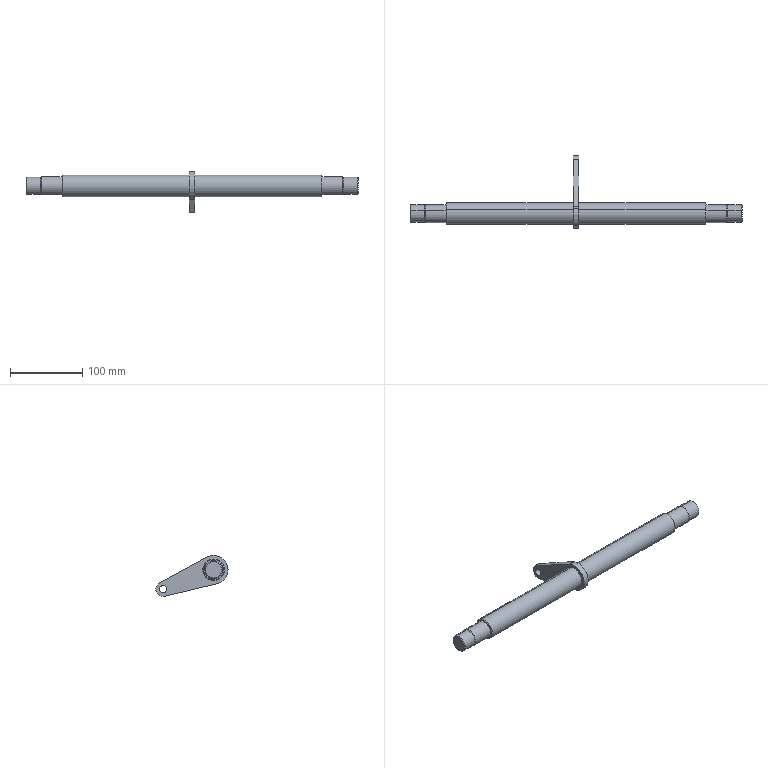Component | SolidWorks | OT-0100-005(RotatingShaft)-1 | 1 solid | 40 faces | box 460 x 99.97 x 57 mm | volume 319935 mm3 | cylinder 18 | cone 12 | plane 10 | commonest cylinder face diameters 30 x4 25 x4 24 x4 40 x3 10 x2 20 x1 | material Plain Carbon Steel
build123d program:
from build123d import *

# Parameters (mm, degrees)
SKETCH4_R           = 12
BOSS_EXTRUDE1_DEPTH = 20
BOSS_EXTRUDE2_START = 20
SKETCH5_R           = 12
BOSS_EXTRUDE2_DEPTH = 20
CHAMFER1_SIZE       = 1
SKETCH6_R           = 5
BOSS_EXTRUDE3_DEPTH = 4


with BuildPart() as part:
    # Sketch1 → Revolve1 (revolve)
    with BuildSketch(Plane(origin=(0, 0, 0), x_dir=(1, 0, 0), z_dir=(0, 1, 0))):
        Polygon((-210, 0), (-210, 11.5), (-209, 12.5), (-180, 12.5), (-180, 14), (-179, 15), (179, 15), (180, 14), (180, 12.5), (209, 12.5), (210, 11.5), (210, 0), align=None)
    revolve(axis=Axis((210, 0, 0), (-1, 0, 0)))

    # Sketch4 → Boss-Extrude1 (add)
    with BuildSketch(Plane(origin=(210, 0, 0), x_dir=(0, 0, -1), z_dir=(1, 0, 0))):
        Circle(SKETCH4_R)
    extrude(amount=BOSS_EXTRUDE1_DEPTH)

    # Sketch5 → Boss-Extrude2 (add)
    with BuildSketch(Plane.ZY.offset(210).offset(BOSS_EXTRUDE2_START)):
        with Locations(Location((0, 0, 0), (0, 0, 180))):
            Circle(SKETCH5_R)
    extrude(amount=-BOSS_EXTRUDE2_DEPTH)

    # Chamfer1
    chamfer1_edges = [part.edges().sort_by_distance(p)[0] for p in [
        (230, 0, 12),
        (-230, 0, 12),
    ]]
    chamfer(chamfer1_edges, length=CHAMFER1_SIZE)

    # Sketch6 → Boss-Extrude3 (add, symmetric)
    with BuildSketch(Plane(origin=(0, 0, 0), x_dir=(0, 0, -1), z_dir=(1, 0, 0))):
        with BuildLine():
            Line((-19.821, 2.667), (-9.911, 76.333))
            ThreePointArc((-9.911, 76.333), (0, 85), (9.911, 76.333))
            Line((9.911, 76.333), (19.821, 2.667))
            ThreePointArc((19.821, 2.667), (0, -20), (-19.821, 2.667))
        make_face()
        with Locations((0, 75)):
            Circle(SKETCH6_R, mode=Mode.SUBTRACT)
    extrude(amount=BOSS_EXTRUDE3_DEPTH, both=True)


solid = part.part

# Placed as in the assembly
solid = solid.moved(Location((200, 35, 0), (-21.097, 0, 0)))
STEP:
#1=COLOUR_RGB('',0.7922,0.8196,0.9333);
#2=FILL_AREA_STYLE_COLOUR('',#1);
#3=FILL_AREA_STYLE('',(#2));
#4=SURFACE_STYLE_FILL_AREA(#3);
#5=SURFACE_SIDE_STYLE('',(#4));
#6=SURFACE_STYLE_USAGE(.BOTH.,#5);
#7=PRESENTATION_STYLE_ASSIGNMENT((#6));
#8=CARTESIAN_POINT('',(8.031,1.591,0.551));
#9=VERTEX_POINT('',#8);
#10=CARTESIAN_POINT('',(8.031,1.165,-0.551));
#11=VERTEX_POINT('',#10);
#12=CARTESIAN_POINT('',(8.031,1.378,0.));
#13=DIRECTION('',(-1.,0.,0.));
#14=DIRECTION('',(0.,-0.3599,-0.933));
#15=AXIS2_PLACEMENT_3D('',#12,#13,#14);
#16=CIRCLE('',#15,0.5906);
#17=EDGE_CURVE('',#9,#11,#16,.T.);
#18=ORIENTED_EDGE('',*,*,#17,.F.);
#19=CARTESIAN_POINT('',(14.921,1.591,0.551));
#20=VERTEX_POINT('',#19);
#21=CARTESIAN_POINT('',(16.142,1.591,0.551));
#22=DIRECTION('',(1.,0.,0.));
#23=VECTOR('',#22,39.37);
#24=LINE('',#21,#23);
#25=EDGE_CURVE('',#9,#20,#24,.T.);
#26=ORIENTED_EDGE('',*,*,#25,.T.);
#27=CARTESIAN_POINT('',(14.921,1.165,-0.551));
#28=VERTEX_POINT('',#27);
#29=CARTESIAN_POINT('',(14.921,1.378,0.));
#30=DIRECTION('',(1.,0.,0.));
#31=DIRECTION('',(0.,-0.3599,-0.933));
#32=AXIS2_PLACEMENT_3D('',#29,#30,#31);
#33=CIRCLE('',#32,0.5906);
#34=EDGE_CURVE('',#28,#20,#33,.T.);
#35=ORIENTED_EDGE('',*,*,#34,.F.);
#36=CARTESIAN_POINT('',(16.142,1.165,-0.551));
#37=DIRECTION('',(1.,0.,0.));
#38=VECTOR('',#37,39.37);
#39=LINE('',#36,#38);
#40=EDGE_CURVE('',#11,#28,#39,.T.);
#41=ORIENTED_EDGE('',*,*,#40,.F.);
#42=EDGE_LOOP('',(#18,#26,#35,#41));
#43=FACE_OUTER_BOUND('',#42,.T.);
#44=CARTESIAN_POINT('',(16.142,1.378,0.));
#45=DIRECTION('',(1.,0.,0.));
#46=DIRECTION('',(0.,-0.3599,-0.933));
#47=AXIS2_PLACEMENT_3D('',#44,#45,#46);
#48=CYLINDRICAL_SURFACE('',#47,0.5906);
#49=ADVANCED_FACE('',(#43),#48,.T.);
#50=CARTESIAN_POINT('',(14.961,1.18,-0.5142));
#51=VERTEX_POINT('',#50);
#52=CARTESIAN_POINT('',(14.961,1.576,0.5142));
#53=VERTEX_POINT('',#52);
#54=CARTESIAN_POINT('',(14.961,1.378,0.));
#55=DIRECTION('',(1.,0.,0.));
#56=DIRECTION('',(0.,-0.3599,-0.933));
#57=AXIS2_PLACEMENT_3D('',#54,#55,#56);
#58=CIRCLE('',#57,0.5512);
#59=EDGE_CURVE('',#51,#53,#58,.T.);
#60=ORIENTED_EDGE('',*,*,#59,.F.);
#61=CARTESIAN_POINT('',(14.961,1.18,-0.5142));
#62=DIRECTION('',(-0.7071,-0.2545,-0.6597));
#63=VECTOR('',#62,39.37);
#64=LINE('',#61,#63);
#65=EDGE_CURVE('',#51,#28,#64,.T.);
#66=ORIENTED_EDGE('',*,*,#65,.T.);
#67=ORIENTED_EDGE('',*,*,#34,.T.);
#68=CARTESIAN_POINT('',(14.961,1.576,0.5142));
#69=DIRECTION('',(-0.7071,0.2545,0.6597));
#70=VECTOR('',#69,39.37);
#71=LINE('',#68,#70);
#72=EDGE_CURVE('',#53,#20,#71,.T.);
#73=ORIENTED_EDGE('',*,*,#72,.F.);
#74=EDGE_LOOP('',(#60,#66,#67,#73));
#75=FACE_OUTER_BOUND('',#74,.T.);
#76=CARTESIAN_POINT('',(14.961,1.378,0.));
#77=DIRECTION('',(-1.,0.,0.));
#78=DIRECTION('',(0.,0.3599,0.933));
#79=AXIS2_PLACEMENT_3D('',#76,#77,#78);
#80=CONICAL_SURFACE('',#79,0.5512,0.7854);
#81=ADVANCED_FACE('',(#75),#80,.T.);
#82=CARTESIAN_POINT('',(14.961,1.201,-0.4591));
#83=VERTEX_POINT('',#82);
#84=CARTESIAN_POINT('',(14.961,1.555,0.4591));
#85=VERTEX_POINT('',#84);
#86=CARTESIAN_POINT('',(14.961,1.378,0.));
#87=DIRECTION('',(1.,0.,0.));
#88=DIRECTION('',(0.,-0.3599,-0.933));
#89=AXIS2_PLACEMENT_3D('',#86,#87,#88);
#90=CIRCLE('',#89,0.4921);
#91=EDGE_CURVE('',#83,#85,#90,.T.);
#92=ORIENTED_EDGE('',*,*,#91,.T.);
#93=CARTESIAN_POINT('',(16.102,1.555,0.4591));
#94=VERTEX_POINT('',#93);
#95=CARTESIAN_POINT('',(16.142,1.555,0.4591));
#96=DIRECTION('',(1.,0.,0.));
#97=VECTOR('',#96,39.37);
#98=LINE('',#95,#97);
#99=EDGE_CURVE('',#85,#94,#98,.T.);
#100=ORIENTED_EDGE('',*,*,#99,.T.);
#101=CARTESIAN_POINT('',(16.102,1.201,-0.4591));
#102=VERTEX_POINT('',#101);
#103=CARTESIAN_POINT('',(16.102,1.378,0.));
#104=DIRECTION('',(1.,0.,0.));
#105=DIRECTION('',(0.,-0.3599,-0.933));
#106=AXIS2_PLACEMENT_3D('',#103,#104,#105);
#107=CIRCLE('',#106,0.4921);
#108=EDGE_CURVE('',#102,#94,#107,.T.);
#109=ORIENTED_EDGE('',*,*,#108,.F.);
#110=CARTESIAN_POINT('',(16.142,1.201,-0.4591));
#111=DIRECTION('',(1.,0.,0.));
#112=VECTOR('',#111,39.37);
#113=LINE('',#110,#112);
#114=EDGE_CURVE('',#83,#102,#113,.T.);
#115=ORIENTED_EDGE('',*,*,#114,.F.);
#116=EDGE_LOOP('',(#92,#100,#109,#115));
#117=FACE_OUTER_BOUND('',#116,.T.);
#118=CARTESIAN_POINT('',(16.142,1.378,0.));
#119=DIRECTION('',(1.,0.,0.));
#120=DIRECTION('',(0.,-0.3599,-0.933));
#121=AXIS2_PLACEMENT_3D('',#118,#119,#120);
#122=CYLINDRICAL_SURFACE('',#121,0.4921);
#123=ADVANCED_FACE('',(#117),#122,.T.);
#124=CARTESIAN_POINT('',(16.142,1.215,-0.4224));
#125=VERTEX_POINT('',#124);
#126=CARTESIAN_POINT('',(16.142,1.541,0.4224));
#127=VERTEX_POINT('',#126);
#128=CARTESIAN_POINT('',(16.142,1.378,0.));
#129=DIRECTION('',(1.,0.,0.));
#130=DIRECTION('',(0.,-0.3599,-0.933));
#131=AXIS2_PLACEMENT_3D('',#128,#129,#130);
#132=CIRCLE('',#131,0.4528);
#133=EDGE_CURVE('',#125,#127,#132,.T.);
#134=ORIENTED_EDGE('',*,*,#133,.F.);
#135=CARTESIAN_POINT('',(16.142,1.215,-0.4224));
#136=DIRECTION('',(-0.7071,-0.2545,-0.6597));
#137=VECTOR('',#136,39.37);
#138=LINE('',#135,#137);
#139=EDGE_CURVE('',#125,#102,#138,.T.);
#140=ORIENTED_EDGE('',*,*,#139,.T.);
#141=ORIENTED_EDGE('',*,*,#108,.T.);
#142=CARTESIAN_POINT('',(16.142,1.541,0.4224));
#143=DIRECTION('',(-0.7071,0.2545,0.6597));
#144=VECTOR('',#143,39.37);
#145=LINE('',#142,#144);
#146=EDGE_CURVE('',#127,#94,#145,.T.);
#147=ORIENTED_EDGE('',*,*,#146,.F.);
#148=EDGE_LOOP('',(#134,#140,#141,#147));
#149=FACE_OUTER_BOUND('',#148,.T.);
#150=CARTESIAN_POINT('',(16.142,1.378,0.));
#151=DIRECTION('',(-1.,0.,0.));
#152=DIRECTION('',(0.,0.3599,0.933));
#153=AXIS2_PLACEMENT_3D('',#150,#151,#152);
#154=CONICAL_SURFACE('',#153,0.4528,0.7854);
#155=ADVANCED_FACE('',(#149),#154,.T.);
#156=CARTESIAN_POINT('',(16.89,1.548,0.4408));
#157=VERTEX_POINT('',#156);
#158=CARTESIAN_POINT('',(16.89,1.208,-0.4408));
#159=VERTEX_POINT('',#158);
#160=CARTESIAN_POINT('',(16.89,1.378,0.));
#161=DIRECTION('',(-1.,0.,0.));
#162=DIRECTION('',(0.,-0.3599,-0.933));
#163=AXIS2_PLACEMENT_3D('',#160,#161,#162);
#164=CIRCLE('',#163,0.4724);
#165=EDGE_CURVE('',#157,#159,#164,.T.);
#166=ORIENTED_EDGE('',*,*,#165,.T.);
#167=CARTESIAN_POINT('',(16.142,1.208,-0.4408));
#168=VERTEX_POINT('',#167);
#169=CARTESIAN_POINT('',(16.929,1.208,-0.4408));
#170=DIRECTION('',(-1.,0.,0.));
#171=VECTOR('',#170,39.37);
#172=LINE('',#169,#171);
#173=EDGE_CURVE('',#159,#168,#172,.T.);
#174=ORIENTED_EDGE('',*,*,#173,.T.);
#175=CARTESIAN_POINT('',(16.142,1.548,0.4408));
#176=VERTEX_POINT('',#175);
#177=CARTESIAN_POINT('',(16.142,1.378,0.));
#178=DIRECTION('',(1.,0.,0.));
#179=DIRECTION('',(0.,-0.3599,-0.933));
#180=AXIS2_PLACEMENT_3D('',#177,#178,#179);
#181=CIRCLE('',#180,0.4724);
#182=EDGE_CURVE('',#168,#176,#181,.T.);
#183=ORIENTED_EDGE('',*,*,#182,.T.);
#184=CARTESIAN_POINT('',(16.929,1.548,0.4408));
#185=DIRECTION('',(-1.,0.,0.));
#186=VECTOR('',#185,39.37);
#187=LINE('',#184,#186);
#188=EDGE_CURVE('',#157,#176,#187,.T.);
#189=ORIENTED_EDGE('',*,*,#188,.F.);
#190=EDGE_LOOP('',(#166,#174,#183,#189));
#191=FACE_OUTER_BOUND('',#190,.T.);
#192=CARTESIAN_POINT('',(16.929,1.378,0.));
#193=DIRECTION('',(-1.,0.,0.));
#194=DIRECTION('',(0.,0.3599,0.933));
#195=AXIS2_PLACEMENT_3D('',#192,#193,#194);
#196=CYLINDRICAL_SURFACE('',#195,0.4724);
#197=ADVANCED_FACE('',(#191),#196,.T.);
#198=CARTESIAN_POINT('',(16.929,1.222,-0.404));
#199=VERTEX_POINT('',#198);
#200=CARTESIAN_POINT('',(16.929,1.534,0.404));
#201=VERTEX_POINT('',#200);
#202=CARTESIAN_POINT('',(16.929,1.378,0.));
#203=DIRECTION('',(1.,0.,0.));
#204=DIRECTION('',(0.,-0.3599,-0.933));
#205=AXIS2_PLACEMENT_3D('',#202,#203,#204);
#206=CIRCLE('',#205,0.4331);
#207=EDGE_CURVE('',#199,#201,#206,.T.);
#208=ORIENTED_EDGE('',*,*,#207,.F.);
#209=CARTESIAN_POINT('',(16.929,1.222,-0.404));
#210=DIRECTION('',(-0.7071,-0.2545,-0.6597));
#211=VECTOR('',#210,39.37);
#212=LINE('',#209,#211);
#213=EDGE_CURVE('',#199,#159,#212,.T.);
#214=ORIENTED_EDGE('',*,*,#213,.T.);
#215=ORIENTED_EDGE('',*,*,#165,.F.);
#216=CARTESIAN_POINT('',(16.929,1.534,0.404));
#217=DIRECTION('',(-0.7071,0.2545,0.6597));
#218=VECTOR('',#217,39.37);
#219=LINE('',#216,#218);
#220=EDGE_CURVE('',#201,#157,#219,.T.);
#221=ORIENTED_EDGE('',*,*,#220,.F.);
#222=EDGE_LOOP('',(#208,#214,#215,#221));
#223=FACE_OUTER_BOUND('',#222,.T.);
#224=CARTESIAN_POINT('',(16.929,1.378,0.));
#225=DIRECTION('',(-1.,0.,0.));
#226=DIRECTION('',(0.,0.3599,0.933));
#227=AXIS2_PLACEMENT_3D('',#224,#225,#226);
#228=CONICAL_SURFACE('',#227,0.4331,0.7854);
#229=ADVANCED_FACE('',(#223),#228,.T.);
#230=CARTESIAN_POINT('',(7.717,4.204,-0.8792));
#231=VERTEX_POINT('',#230);
#232=CARTESIAN_POINT('',(7.717,4.062,-1.246));
#233=VERTEX_POINT('',#232);
#234=CARTESIAN_POINT('',(7.717,4.133,-1.063));
#235=DIRECTION('',(1.,0.,0.));
#236=DIRECTION('',(0.,-0.3599,-0.933));
#237=AXIS2_PLACEMENT_3D('',#234,#235,#236);
#238=CIRCLE('',#237,0.1969);
#239=EDGE_CURVE('',#231,#233,#238,.T.);
#240=ORIENTED_EDGE('',*,*,#239,.F.);
#241=CARTESIAN_POINT('',(8.031,4.204,-0.8792));
#242=VERTEX_POINT('',#241);
#243=CARTESIAN_POINT('',(7.717,4.204,-0.8792));
#244=DIRECTION('',(1.,0.,0.));
#245=VECTOR('',#244,39.37);
#246=LINE('',#243,#245);
#247=EDGE_CURVE('',#231,#242,#246,.T.);
#248=ORIENTED_EDGE('',*,*,#247,.T.);
#249=CARTESIAN_POINT('',(8.031,4.062,-1.246));
#250=VERTEX_POINT('',#249);
#251=CARTESIAN_POINT('',(8.031,4.133,-1.063));
#252=DIRECTION('',(1.,0.,0.));
#253=DIRECTION('',(0.,-0.3599,-0.933));
#254=AXIS2_PLACEMENT_3D('',#251,#252,#253);
#255=CIRCLE('',#254,0.1969);
#256=EDGE_CURVE('',#242,#250,#255,.T.);
#257=ORIENTED_EDGE('',*,*,#256,.T.);
#258=CARTESIAN_POINT('',(7.717,4.062,-1.246));
#259=DIRECTION('',(1.,0.,0.));
#260=VECTOR('',#259,39.37);
#261=LINE('',#258,#260);
#262=EDGE_CURVE('',#233,#250,#261,.T.);
#263=ORIENTED_EDGE('',*,*,#262,.F.);
#264=EDGE_LOOP('',(#240,#248,#257,#263));
#265=FACE_OUTER_BOUND('',#264,.T.);
#266=CARTESIAN_POINT('',(7.717,4.133,-1.063));
#267=DIRECTION('',(1.,0.,0.));
#268=DIRECTION('',(0.,-0.3599,-0.933));
#269=AXIS2_PLACEMENT_3D('',#266,#267,#268);
#270=CYLINDRICAL_SURFACE('',#269,0.1969);
#271=ADVANCED_FACE('',(#265),#270,.F.);
#272=CARTESIAN_POINT('',(7.717,1.757,0.6903));
#273=VERTEX_POINT('',#272);
#274=CARTESIAN_POINT('',(7.717,1.661,0.7346));
#275=VERTEX_POINT('',#274);
#276=CARTESIAN_POINT('',(7.717,1.378,0.));
#277=DIRECTION('',(1.,0.,0.));
#278=DIRECTION('',(0.,-0.3599,-0.933));
#279=AXIS2_PLACEMENT_3D('',#276,#277,#278);
#280=CIRCLE('',#279,0.7874);
#281=EDGE_CURVE('',#273,#275,#280,.T.);
#282=ORIENTED_EDGE('',*,*,#281,.T.);
#283=CARTESIAN_POINT('',(8.031,1.661,0.7346));
#284=VERTEX_POINT('',#283);
#285=CARTESIAN_POINT('',(7.717,1.661,0.7346));
#286=DIRECTION('',(1.,0.,0.));
#287=VECTOR('',#286,39.37);
#288=LINE('',#285,#287);
#289=EDGE_CURVE('',#275,#284,#288,.T.);
#290=ORIENTED_EDGE('',*,*,#289,.T.);
#291=CARTESIAN_POINT('',(8.031,1.757,0.6903));
#292=VERTEX_POINT('',#291);
#293=CARTESIAN_POINT('',(8.031,1.378,0.));
#294=DIRECTION('',(1.,0.,0.));
#295=DIRECTION('',(0.,-0.3599,-0.933));
#296=AXIS2_PLACEMENT_3D('',#293,#294,#295);
#297=CIRCLE('',#296,0.7874);
#298=EDGE_CURVE('',#292,#284,#297,.T.);
#299=ORIENTED_EDGE('',*,*,#298,.F.);
#300=CARTESIAN_POINT('',(7.717,1.757,0.6903));
#301=DIRECTION('',(1.,0.,0.));
#302=VECTOR('',#301,39.37);
#303=LINE('',#300,#302);
#304=EDGE_CURVE('',#273,#292,#303,.T.);
#305=ORIENTED_EDGE('',*,*,#304,.F.);
#306=EDGE_LOOP('',(#282,#290,#299,#305));
#307=FACE_OUTER_BOUND('',#306,.T.);
#308=CARTESIAN_POINT('',(7.717,1.378,0.));
#309=DIRECTION('',(1.,0.,0.));
#310=DIRECTION('',(0.,-0.3599,-0.933));
#311=AXIS2_PLACEMENT_3D('',#308,#309,#310);
#312=CYLINDRICAL_SURFACE('',#311,0.7874);
#313=ADVANCED_FACE('',(#307),#312,.T.);
#314=ORIENTED_EDGE('',*,*,#289,.F.);
#315=CARTESIAN_POINT('',(7.717,1.095,-0.7346));
#316=VERTEX_POINT('',#315);
#317=CARTESIAN_POINT('',(7.717,1.378,0.));
#318=DIRECTION('',(1.,0.,0.));
#319=DIRECTION('',(0.,-0.3599,-0.933));
#320=AXIS2_PLACEMENT_3D('',#317,#318,#319);
#321=CIRCLE('',#320,0.7874);
#322=EDGE_CURVE('',#275,#316,#321,.T.);
#323=ORIENTED_EDGE('',*,*,#322,.T.);
#324=CARTESIAN_POINT('',(8.031,1.095,-0.7346));
#325=VERTEX_POINT('',#324);
#326=CARTESIAN_POINT('',(7.717,1.095,-0.7346));
#327=DIRECTION('',(1.,0.,0.));
#328=VECTOR('',#327,39.37);
#329=LINE('',#326,#328);
#330=EDGE_CURVE('',#316,#325,#329,.T.);
#331=ORIENTED_EDGE('',*,*,#330,.T.);
#332=CARTESIAN_POINT('',(8.031,1.378,0.));
#333=DIRECTION('',(1.,0.,0.));
#334=DIRECTION('',(0.,-0.3599,-0.933));
#335=AXIS2_PLACEMENT_3D('',#332,#333,#334);
#336=CIRCLE('',#335,0.7874);
#337=EDGE_CURVE('',#284,#325,#336,.T.);
#338=ORIENTED_EDGE('',*,*,#337,.F.);
#339=EDGE_LOOP('',(#314,#323,#331,#338));
#340=FACE_OUTER_BOUND('',#339,.T.);
#341=CARTESIAN_POINT('',(7.717,1.378,0.));
#342=DIRECTION('',(1.,0.,0.));
#343=DIRECTION('',(0.,-0.3599,-0.933));
#344=AXIS2_PLACEMENT_3D('',#341,#342,#343);
#345=CYLINDRICAL_SURFACE('',#344,0.7874);
#346=ADVANCED_FACE('',(#340),#345,.T.);
#347=CARTESIAN_POINT('',(-1.181,1.534,0.404));
#348=VERTEX_POINT('',#347);
#349=CARTESIAN_POINT('',(-1.181,1.222,-0.404));
#350=VERTEX_POINT('',#349);
#351=CARTESIAN_POINT('',(-1.181,1.378,0.));
#352=DIRECTION('',(-1.,0.,0.));
#353=DIRECTION('',(0.,0.3599,0.933));
#354=AXIS2_PLACEMENT_3D('',#351,#352,#353);
#355=CIRCLE('',#354,0.4331);
#356=EDGE_CURVE('',#348,#350,#355,.T.);
#357=ORIENTED_EDGE('',*,*,#356,.F.);
#358=CARTESIAN_POINT('',(-1.142,1.548,0.4408));
#359=VERTEX_POINT('',#358);
#360=CARTESIAN_POINT('',(-1.181,1.534,0.404));
#361=DIRECTION('',(0.7071,0.2545,0.6597));
#362=VECTOR('',#361,39.37);
#363=LINE('',#360,#362);
#364=EDGE_CURVE('',#348,#359,#363,.T.);
#365=ORIENTED_EDGE('',*,*,#364,.T.);
#366=CARTESIAN_POINT('',(-1.142,1.208,-0.4408));
#367=VERTEX_POINT('',#366);
#368=CARTESIAN_POINT('',(-1.142,1.378,0.));
#369=DIRECTION('',(1.,0.,0.));
#370=DIRECTION('',(0.,0.3599,0.933));
#371=AXIS2_PLACEMENT_3D('',#368,#369,#370);
#372=CIRCLE('',#371,0.4724);
#373=EDGE_CURVE('',#367,#359,#372,.T.);
#374=ORIENTED_EDGE('',*,*,#373,.F.);
#375=CARTESIAN_POINT('',(-1.181,1.222,-0.404));
#376=DIRECTION('',(0.7071,-0.2545,-0.6597));
#377=VECTOR('',#376,39.37);
#378=LINE('',#375,#377);
#379=EDGE_CURVE('',#350,#367,#378,.T.);
#380=ORIENTED_EDGE('',*,*,#379,.F.);
#381=EDGE_LOOP('',(#357,#365,#374,#380));
#382=FACE_OUTER_BOUND('',#381,.T.);
#383=CARTESIAN_POINT('',(-1.181,1.378,0.));
#384=DIRECTION('',(1.,0.,0.));
#385=DIRECTION('',(0.,-0.3599,-0.933));
#386=AXIS2_PLACEMENT_3D('',#383,#384,#385);
#387=CONICAL_SURFACE('',#386,0.4331,0.7854);
#388=ADVANCED_FACE('',(#382),#387,.T.);
#389=ORIENTED_EDGE('',*,*,#373,.T.);
#390=CARTESIAN_POINT('',(-0.3937,1.548,0.4408));
#391=VERTEX_POINT('',#390);
#392=CARTESIAN_POINT('',(-1.181,1.548,0.4408));
#393=DIRECTION('',(1.,0.,0.));
#394=VECTOR('',#393,39.37);
#395=LINE('',#392,#394);
#396=EDGE_CURVE('',#359,#391,#395,.T.);
#397=ORIENTED_EDGE('',*,*,#396,.T.);
#398=CARTESIAN_POINT('',(-0.3937,1.208,-0.4408));
#399=VERTEX_POINT('',#398);
#400=CARTESIAN_POINT('',(-0.3937,1.378,0.));
#401=DIRECTION('',(-1.,0.,0.));
#402=DIRECTION('',(0.,0.3599,0.933));
#403=AXIS2_PLACEMENT_3D('',#400,#401,#402);
#404=CIRCLE('',#403,0.4724);
#405=EDGE_CURVE('',#391,#399,#404,.T.);
#406=ORIENTED_EDGE('',*,*,#405,.T.);
#407=CARTESIAN_POINT('',(-1.181,1.208,-0.4408));
#408=DIRECTION('',(1.,0.,0.));
#409=VECTOR('',#408,39.37);
#410=LINE('',#407,#409);
#411=EDGE_CURVE('',#367,#399,#410,.T.);
#412=ORIENTED_EDGE('',*,*,#411,.F.);
#413=EDGE_LOOP('',(#389,#397,#406,#412));
#414=FACE_OUTER_BOUND('',#413,.T.);
#415=CARTESIAN_POINT('',(-1.181,1.378,0.));
#416=DIRECTION('',(1.,0.,0.));
#417=DIRECTION('',(0.,-0.3599,-0.933));
#418=AXIS2_PLACEMENT_3D('',#415,#416,#417);
#419=CYLINDRICAL_SURFACE('',#418,0.4724);
#420=ADVANCED_FACE('',(#414),#419,.T.);
#421=CARTESIAN_POINT('',(0.7874,1.18,-0.5142));
#422=VERTEX_POINT('',#421);
#423=CARTESIAN_POINT('',(0.7874,1.576,0.5142));
#424=VERTEX_POINT('',#423);
#425=CARTESIAN_POINT('',(0.7874,1.378,0.));
#426=DIRECTION('',(1.,0.,0.));
#427=DIRECTION('',(0.,-0.3599,-0.933));
#428=AXIS2_PLACEMENT_3D('',#425,#426,#427);
#429=CIRCLE('',#428,0.5512);
#430=EDGE_CURVE('',#422,#424,#429,.T.);
#431=ORIENTED_EDGE('',*,*,#430,.T.);
#432=CARTESIAN_POINT('',(0.8268,1.591,0.551));
#433=VERTEX_POINT('',#432);
#434=CARTESIAN_POINT('',(0.8268,1.591,0.551));
#435=DIRECTION('',(0.7071,0.2545,0.6597));
#436=VECTOR('',#435,39.37);
#437=LINE('',#434,#436);
#438=EDGE_CURVE('',#424,#433,#437,.T.);
#439=ORIENTED_EDGE('',*,*,#438,.T.);
#440=CARTESIAN_POINT('',(0.8268,1.165,-0.551));
#441=VERTEX_POINT('',#440);
#442=CARTESIAN_POINT('',(0.8268,1.378,0.));
#443=DIRECTION('',(1.,0.,0.));
#444=DIRECTION('',(0.,-0.3599,-0.933));
#445=AXIS2_PLACEMENT_3D('',#442,#443,#444);
#446=CIRCLE('',#445,0.5906);
#447=EDGE_CURVE('',#441,#433,#446,.T.);
#448=ORIENTED_EDGE('',*,*,#447,.F.);
#449=CARTESIAN_POINT('',(0.8268,1.165,-0.551));
#450=DIRECTION('',(0.7071,-0.2545,-0.6597));
#451=VECTOR('',#450,39.37);
#452=LINE('',#449,#451);
#453=EDGE_CURVE('',#422,#441,#452,.T.);
#454=ORIENTED_EDGE('',*,*,#453,.F.);
#455=EDGE_LOOP('',(#431,#439,#448,#454));
#456=FACE_OUTER_BOUND('',#455,.T.);
#457=CARTESIAN_POINT('',(0.8268,1.378,0.));
#458=DIRECTION('',(1.,0.,0.));
#459=DIRECTION('',(0.,-0.3599,-0.933));
#460=AXIS2_PLACEMENT_3D('',#457,#458,#459);
#461=CONICAL_SURFACE('',#460,0.5906,0.7854);
#462=ADVANCED_FACE('',(#456),#461,.T.);
#463=CARTESIAN_POINT('',(-0.3543,1.201,-0.4591));
#464=VERTEX_POINT('',#463);
#465=CARTESIAN_POINT('',(-0.3543,1.555,0.4591));
#466=VERTEX_POINT('',#465);
#467=CARTESIAN_POINT('',(-0.3543,1.378,0.));
#468=DIRECTION('',(1.,0.,0.));
#469=DIRECTION('',(0.,-0.3599,-0.933));
#470=AXIS2_PLACEMENT_3D('',#467,#468,#469);
#471=CIRCLE('',#470,0.4921);
#472=EDGE_CURVE('',#464,#466,#471,.T.);
#473=ORIENTED_EDGE('',*,*,#472,.T.);
#474=CARTESIAN_POINT('',(0.7874,1.555,0.4591));
#475=VERTEX_POINT('',#474);
#476=CARTESIAN_POINT('',(16.142,1.555,0.4591));
#477=DIRECTION('',(1.,0.,0.));
#478=VECTOR('',#477,39.37);
#479=LINE('',#476,#478);
#480=EDGE_CURVE('',#466,#475,#479,.T.);
#481=ORIENTED_EDGE('',*,*,#480,.T.);
#482=CARTESIAN_POINT('',(0.7874,1.201,-0.4591));
#483=VERTEX_POINT('',#482);
#484=CARTESIAN_POINT('',(0.7874,1.378,0.));
#485=DIRECTION('',(1.,0.,0.));
#486=DIRECTION('',(0.,-0.3599,-0.933));
#487=AXIS2_PLACEMENT_3D('',#484,#485,#486);
#488=CIRCLE('',#487,0.4921);
#489=EDGE_CURVE('',#483,#475,#488,.T.);
#490=ORIENTED_EDGE('',*,*,#489,.F.);
#491=CARTESIAN_POINT('',(16.142,1.201,-0.4591));
#492=DIRECTION('',(1.,0.,0.));
#493=VECTOR('',#492,39.37);
#494=LINE('',#491,#493);
#495=EDGE_CURVE('',#464,#483,#494,.T.);
#496=ORIENTED_EDGE('',*,*,#495,.F.);
#497=EDGE_LOOP('',(#473,#481,#490,#496));
#498=FACE_OUTER_BOUND('',#497,.T.);
#499=CARTESIAN_POINT('',(16.142,1.378,0.));
#500=DIRECTION('',(1.,0.,0.));
#501=DIRECTION('',(0.,-0.3599,-0.933));
#502=AXIS2_PLACEMENT_3D('',#499,#500,#501);
#503=CYLINDRICAL_SURFACE('',#502,0.4921);
#504=ADVANCED_FACE('',(#498),#503,.T.);
#505=CARTESIAN_POINT('',(-0.3937,1.215,-0.4224));
#506=VERTEX_POINT('',#505);
#507=CARTESIAN_POINT('',(-0.3937,1.541,0.4224));
#508=VERTEX_POINT('',#507);
#509=CARTESIAN_POINT('',(-0.3937,1.378,0.));
#510=DIRECTION('',(1.,0.,0.));
#511=DIRECTION('',(0.,0.3599,0.933));
#512=AXIS2_PLACEMENT_3D('',#509,#510,#511);
#513=CIRCLE('',#512,0.4528);
#514=EDGE_CURVE('',#506,#508,#513,.T.);
#515=ORIENTED_EDGE('',*,*,#514,.T.);
#516=CARTESIAN_POINT('',(-0.3543,1.555,0.4591));
#517=DIRECTION('',(0.7071,0.2545,0.6597));
#518=VECTOR('',#517,39.37);
#519=LINE('',#516,#518);
#520=EDGE_CURVE('',#508,#466,#519,.T.);
#521=ORIENTED_EDGE('',*,*,#520,.T.);
#522=ORIENTED_EDGE('',*,*,#472,.F.);
#523=CARTESIAN_POINT('',(-0.3543,1.201,-0.4591));
#524=DIRECTION('',(0.7071,-0.2545,-0.6597));
#525=VECTOR('',#524,39.37);
#526=LINE('',#523,#525);
#527=EDGE_CURVE('',#506,#464,#526,.T.);
#528=ORIENTED_EDGE('',*,*,#527,.F.);
#529=EDGE_LOOP('',(#515,#521,#522,#528));
#530=FACE_OUTER_BOUND('',#529,.T.);
#531=CARTESIAN_POINT('',(-0.3543,1.378,0.));
#532=DIRECTION('',(1.,0.,0.));
#533=DIRECTION('',(0.,-0.3599,-0.933));
#534=AXIS2_PLACEMENT_3D('',#531,#532,#533);
#535=CONICAL_SURFACE('',#534,0.4921,0.7854);
#536=ADVANCED_FACE('',(#530),#535,.T.);
#537=ORIENTED_EDGE('',*,*,#447,.T.);
#538=CARTESIAN_POINT('',(7.717,1.591,0.551));
#539=VERTEX_POINT('',#538);
#540=CARTESIAN_POINT('',(16.142,1.591,0.551));
#541=DIRECTION('',(1.,0.,0.));
#542=VECTOR('',#541,39.37);
#543=LINE('',#540,#542);
#544=EDGE_CURVE('',#433,#539,#543,.T.);
#545=ORIENTED_EDGE('',*,*,#544,.T.);
#546=CARTESIAN_POINT('',(7.717,1.165,-0.551));
#547=VERTEX_POINT('',#546);
#548=CARTESIAN_POINT('',(7.717,1.378,0.));
#549=DIRECTION('',(-1.,0.,0.));
#550=DIRECTION('',(0.,-0.3599,-0.933));
#551=AXIS2_PLACEMENT_3D('',#548,#549,#550);
#552=CIRCLE('',#551,0.5906);
#553=EDGE_CURVE('',#539,#547,#552,.T.);
#554=ORIENTED_EDGE('',*,*,#553,.T.);
#555=CARTESIAN_POINT('',(16.142,1.165,-0.551));
#556=DIRECTION('',(1.,0.,0.));
#557=VECTOR('',#556,39.37);
#558=LINE('',#555,#557);
#559=EDGE_CURVE('',#441,#547,#558,.T.);
#560=ORIENTED_EDGE('',*,*,#559,.F.);
#561=EDGE_LOOP('',(#537,#545,#554,#560));
#562=FACE_OUTER_BOUND('',#561,.T.);
#563=CARTESIAN_POINT('',(16.142,1.378,0.));
#564=DIRECTION('',(1.,0.,0.));
#565=DIRECTION('',(0.,-0.3599,-0.933));
#566=AXIS2_PLACEMENT_3D('',#563,#564,#565);
#567=CYLINDRICAL_SURFACE('',#566,0.5906);
#568=ADVANCED_FACE('',(#562),#567,.T.);
#569=ORIENTED_EDGE('',*,*,#544,.F.);
#570=CARTESIAN_POINT('',(0.8268,1.378,0.));
#571=DIRECTION('',(1.,0.,0.));
#572=DIRECTION('',(0.,-0.3599,-0.933));
#573=AXIS2_PLACEMENT_3D('',#570,#571,#572);
#574=CIRCLE('',#573,0.5906);
#575=EDGE_CURVE('',#433,#441,#574,.T.);
#576=ORIENTED_EDGE('',*,*,#575,.T.);
#577=ORIENTED_EDGE('',*,*,#559,.T.);
#578=CARTESIAN_POINT('',(7.717,1.378,0.));
#579=DIRECTION('',(-1.,0.,0.));
#580=DIRECTION('',(0.,-0.3599,-0.933));
#581=AXIS2_PLACEMENT_3D('',#578,#579,#580);
#582=CIRCLE('',#581,0.5906);
#583=EDGE_CURVE('',#547,#539,#582,.T.);
#584=ORIENTED_EDGE('',*,*,#583,.T.);
#585=EDGE_LOOP('',(#569,#576,#577,#584));
#586=FACE_OUTER_BOUND('',#585,.T.);
#587=CARTESIAN_POINT('',(16.142,1.378,0.));
#588=DIRECTION('',(1.,0.,0.));
#589=DIRECTION('',(0.,-0.3599,-0.933));
#590=AXIS2_PLACEMENT_3D('',#587,#588,#589);
#591=CYLINDRICAL_SURFACE('',#590,0.5906);
#592=ADVANCED_FACE('',(#586),#591,.T.);
#593=ORIENTED_EDGE('',*,*,#520,.F.);
#594=CARTESIAN_POINT('',(-0.3937,1.378,0.));
#595=DIRECTION('',(1.,0.,0.));
#596=DIRECTION('',(0.,0.3599,0.933));
#597=AXIS2_PLACEMENT_3D('',#594,#595,#596);
#598=CIRCLE('',#597,0.4528);
#599=EDGE_CURVE('',#508,#506,#598,.T.);
#600=ORIENTED_EDGE('',*,*,#599,.T.);
#601=ORIENTED_EDGE('',*,*,#527,.T.);
#602=CARTESIAN_POINT('',(-0.3543,1.378,0.));
#603=DIRECTION('',(1.,0.,0.));
#604=DIRECTION('',(0.,-0.3599,-0.933));
#605=AXIS2_PLACEMENT_3D('',#602,#603,#604);
#606=CIRCLE('',#605,0.4921);
#607=EDGE_CURVE('',#466,#464,#606,.T.);
#608=ORIENTED_EDGE('',*,*,#607,.F.);
#609=EDGE_LOOP('',(#593,#600,#601,#608));
#610=FACE_OUTER_BOUND('',#609,.T.);
#611=CARTESIAN_POINT('',(-0.3543,1.378,0.));
#612=DIRECTION('',(1.,0.,0.));
#613=DIRECTION('',(0.,-0.3599,-0.933));
#614=AXIS2_PLACEMENT_3D('',#611,#612,#613);
#615=CONICAL_SURFACE('',#614,0.4921,0.7854);
#616=ADVANCED_FACE('',(#610),#615,.T.);
#617=ORIENTED_EDGE('',*,*,#480,.F.);
#618=ORIENTED_EDGE('',*,*,#607,.T.);
#619=ORIENTED_EDGE('',*,*,#495,.T.);
#620=CARTESIAN_POINT('',(0.7874,1.378,0.));
#621=DIRECTION('',(1.,0.,0.));
#622=DIRECTION('',(0.,-0.3599,-0.933));
#623=AXIS2_PLACEMENT_3D('',#620,#621,#622);
#624=CIRCLE('',#623,0.4921);
#625=EDGE_CURVE('',#475,#483,#624,.T.);
#626=ORIENTED_EDGE('',*,*,#625,.F.);
#627=EDGE_LOOP('',(#617,#618,#619,#626));
#628=FACE_OUTER_BOUND('',#627,.T.);
#629=CARTESIAN_POINT('',(16.142,1.378,0.));
#630=DIRECTION('',(1.,0.,0.));
#631=DIRECTION('',(0.,-0.3599,-0.933));
#632=AXIS2_PLACEMENT_3D('',#629,#630,#631);
#633=CYLINDRICAL_SURFACE('',#632,0.4921);
#634=ADVANCED_FACE('',(#628),#633,.T.);
#635=ORIENTED_EDGE('',*,*,#489,.T.);
#636=ORIENTED_EDGE('',*,*,#625,.T.);
#637=EDGE_LOOP('',(#635,#636));
#638=FACE_BOUND('',#637,.T.);
#639=ORIENTED_EDGE('',*,*,#430,.F.);
#640=CARTESIAN_POINT('',(0.7874,1.378,0.));
#641=DIRECTION('',(1.,0.,0.));
#642=DIRECTION('',(0.,-0.3599,-0.933));
#643=AXIS2_PLACEMENT_3D('',#640,#641,#642);
#644=CIRCLE('',#643,0.5512);
#645=EDGE_CURVE('',#424,#422,#644,.T.);
#646=ORIENTED_EDGE('',*,*,#645,.F.);
#647=EDGE_LOOP('',(#639,#646));
#648=FACE_OUTER_BOUND('',#647,.T.);
#649=CARTESIAN_POINT('',(0.7874,1.201,-0.4591));
#650=DIRECTION('',(-1.,0.,0.));
#651=DIRECTION('',(0.,0.3599,0.933));
#652=AXIS2_PLACEMENT_3D('',#649,#650,#651);
#653=PLANE('',#652);
#654=ADVANCED_FACE('',(#638,#648),#653,.T.);
#655=ORIENTED_EDGE('',*,*,#438,.F.);
#656=ORIENTED_EDGE('',*,*,#645,.T.);
#657=ORIENTED_EDGE('',*,*,#453,.T.);
#658=ORIENTED_EDGE('',*,*,#575,.F.);
#659=EDGE_LOOP('',(#655,#656,#657,#658));
#660=FACE_OUTER_BOUND('',#659,.T.);
#661=CARTESIAN_POINT('',(0.8268,1.378,0.));
#662=DIRECTION('',(1.,0.,0.));
#663=DIRECTION('',(0.,-0.3599,-0.933));
#664=AXIS2_PLACEMENT_3D('',#661,#662,#663);
#665=CONICAL_SURFACE('',#664,0.5906,0.7854);
#666=ADVANCED_FACE('',(#660),#665,.T.);
#667=ORIENTED_EDGE('',*,*,#396,.F.);
#668=CARTESIAN_POINT('',(-1.142,1.378,0.));
#669=DIRECTION('',(1.,0.,0.));
#670=DIRECTION('',(0.,0.3599,0.933));
#671=AXIS2_PLACEMENT_3D('',#668,#669,#670);
#672=CIRCLE('',#671,0.4724);
#673=EDGE_CURVE('',#359,#367,#672,.T.);
#674=ORIENTED_EDGE('',*,*,#673,.T.);
#675=ORIENTED_EDGE('',*,*,#411,.T.);
#676=CARTESIAN_POINT('',(-0.3937,1.378,0.));
#677=DIRECTION('',(-1.,0.,0.));
#678=DIRECTION('',(0.,0.3599,0.933));
#679=AXIS2_PLACEMENT_3D('',#676,#677,#678);
#680=CIRCLE('',#679,0.4724);
#681=EDGE_CURVE('',#399,#391,#680,.T.);
#682=ORIENTED_EDGE('',*,*,#681,.T.);
#683=EDGE_LOOP('',(#667,#674,#675,#682));
#684=FACE_OUTER_BOUND('',#683,.T.);
#685=CARTESIAN_POINT('',(-1.181,1.378,0.));
#686=DIRECTION('',(1.,0.,0.));
#687=DIRECTION('',(0.,-0.3599,-0.933));
#688=AXIS2_PLACEMENT_3D('',#685,#686,#687);
#689=CYLINDRICAL_SURFACE('',#688,0.4724);
#690=ADVANCED_FACE('',(#684),#689,.T.);
#691=CARTESIAN_POINT('',(-1.181,1.378,0.));
#692=DIRECTION('',(-1.,0.,0.));
#693=DIRECTION('',(0.,0.3599,0.933));
#694=AXIS2_PLACEMENT_3D('',#691,#692,#693);
#695=CIRCLE('',#694,0.4331);
#696=EDGE_CURVE('',#350,#348,#695,.T.);
#697=ORIENTED_EDGE('',*,*,#696,.T.);
#698=ORIENTED_EDGE('',*,*,#356,.T.);
#699=EDGE_LOOP('',(#697,#698));
#700=FACE_OUTER_BOUND('',#699,.T.);
#701=CARTESIAN_POINT('',(-1.181,1.378,0.));
#702=DIRECTION('',(-1.,0.,0.));
#703=DIRECTION('',(0.,0.3599,0.933));
#704=AXIS2_PLACEMENT_3D('',#701,#702,#703);
#705=PLANE('',#704);
#706=ADVANCED_FACE('',(#700),#705,.T.);
#707=ORIENTED_EDGE('',*,*,#514,.F.);
#708=ORIENTED_EDGE('',*,*,#599,.F.);
#709=EDGE_LOOP('',(#707,#708));
#710=FACE_BOUND('',#709,.T.);
#711=ORIENTED_EDGE('',*,*,#681,.F.);
#712=ORIENTED_EDGE('',*,*,#405,.F.);
#713=EDGE_LOOP('',(#711,#712));
#714=FACE_OUTER_BOUND('',#713,.T.);
#715=CARTESIAN_POINT('',(-0.3937,1.378,0.));
#716=DIRECTION('',(-1.,0.,0.));
#717=DIRECTION('',(0.,0.3599,0.933));
#718=AXIS2_PLACEMENT_3D('',#715,#716,#717);
#719=PLANE('',#718);
#720=ADVANCED_FACE('',(#710,#714),#719,.F.);
#721=ORIENTED_EDGE('',*,*,#364,.F.);
#722=ORIENTED_EDGE('',*,*,#696,.F.);
#723=ORIENTED_EDGE('',*,*,#379,.T.);
#724=ORIENTED_EDGE('',*,*,#673,.F.);
#725=EDGE_LOOP('',(#721,#722,#723,#724));
#726=FACE_OUTER_BOUND('',#725,.T.);
#727=CARTESIAN_POINT('',(-1.181,1.378,0.));
#728=DIRECTION('',(1.,0.,0.));
#729=DIRECTION('',(0.,-0.3599,-0.933));
#730=AXIS2_PLACEMENT_3D('',#727,#728,#729);
#731=CONICAL_SURFACE('',#730,0.4331,0.7854);
#732=ADVANCED_FACE('',(#726),#731,.T.);
#733=ORIENTED_EDGE('',*,*,#330,.F.);
#734=CARTESIAN_POINT('',(7.717,1.195,-0.7659));
#735=VERTEX_POINT('',#734);
#736=CARTESIAN_POINT('',(7.717,1.378,0.));
#737=DIRECTION('',(1.,0.,0.));
#738=DIRECTION('',(0.,-0.3599,-0.933));
#739=AXIS2_PLACEMENT_3D('',#736,#737,#738);
#740=CIRCLE('',#739,0.7874);
#741=EDGE_CURVE('',#316,#735,#740,.T.);
#742=ORIENTED_EDGE('',*,*,#741,.T.);
#743=CARTESIAN_POINT('',(8.031,1.195,-0.7659));
#744=VERTEX_POINT('',#743);
#745=CARTESIAN_POINT('',(7.717,1.195,-0.7659));
#746=DIRECTION('',(1.,0.,0.));
#747=VECTOR('',#746,39.37);
#748=LINE('',#745,#747);
#749=EDGE_CURVE('',#735,#744,#748,.T.);
#750=ORIENTED_EDGE('',*,*,#749,.T.);
#751=CARTESIAN_POINT('',(8.031,1.378,0.));
#752=DIRECTION('',(1.,0.,0.));
#753=DIRECTION('',(0.,-0.3599,-0.933));
#754=AXIS2_PLACEMENT_3D('',#751,#752,#753);
#755=CIRCLE('',#754,0.7874);
#756=EDGE_CURVE('',#325,#744,#755,.T.);
#757=ORIENTED_EDGE('',*,*,#756,.F.);
#758=EDGE_LOOP('',(#733,#742,#750,#757));
#759=FACE_OUTER_BOUND('',#758,.T.);
#760=CARTESIAN_POINT('',(7.717,1.378,0.));
#761=DIRECTION('',(1.,0.,0.));
#762=DIRECTION('',(0.,-0.3599,-0.933));
#763=AXIS2_PLACEMENT_3D('',#760,#761,#762);
#764=CYLINDRICAL_SURFACE('',#763,0.7874);
#765=ADVANCED_FACE('',(#759),#764,.T.);
#766=CARTESIAN_POINT('',(8.031,4.322,-0.7177));
#767=VERTEX_POINT('',#766);
#768=CARTESIAN_POINT('',(8.031,1.757,0.6903));
#769=DIRECTION('',(0.,-0.8767,0.4811));
#770=VECTOR('',#769,39.37);
#771=LINE('',#768,#770);
#772=EDGE_CURVE('',#767,#292,#771,.T.);
#773=ORIENTED_EDGE('',*,*,#772,.F.);
#774=CARTESIAN_POINT('',(7.717,4.322,-0.7177));
#775=VERTEX_POINT('',#774);
#776=CARTESIAN_POINT('',(7.717,4.322,-0.7177));
#777=DIRECTION('',(1.,0.,0.));
#778=VECTOR('',#777,39.37);
#779=LINE('',#776,#778);
#780=EDGE_CURVE('',#775,#767,#779,.T.);
#781=ORIENTED_EDGE('',*,*,#780,.F.);
#782=CARTESIAN_POINT('',(7.717,1.757,0.6903));
#783=DIRECTION('',(0.,-0.8767,0.4811));
#784=VECTOR('',#783,39.37);
#785=LINE('',#782,#784);
#786=EDGE_CURVE('',#775,#273,#785,.T.);
#787=ORIENTED_EDGE('',*,*,#786,.T.);
#788=ORIENTED_EDGE('',*,*,#304,.T.);
#789=EDGE_LOOP('',(#773,#781,#787,#788));
#790=FACE_OUTER_BOUND('',#789,.T.);
#791=CARTESIAN_POINT('',(7.717,1.757,0.6903));
#792=DIRECTION('',(0.,0.4811,0.8767));
#793=DIRECTION('',(0.,-0.8767,0.4811));
#794=AXIS2_PLACEMENT_3D('',#791,#792,#793);
#795=PLANE('',#794);
#796=ADVANCED_FACE('',(#790),#795,.T.);
#797=CARTESIAN_POINT('',(8.031,4.041,-1.446));
#798=VERTEX_POINT('',#797);
#799=CARTESIAN_POINT('',(8.031,4.133,-1.063));
#800=DIRECTION('',(1.,0.,0.));
#801=DIRECTION('',(0.,-0.3599,-0.933));
#802=AXIS2_PLACEMENT_3D('',#799,#800,#801);
#803=CIRCLE('',#802,0.3937);
#804=EDGE_CURVE('',#798,#767,#803,.T.);
#805=ORIENTED_EDGE('',*,*,#804,.F.);
#806=CARTESIAN_POINT('',(7.717,4.041,-1.446));
#807=VERTEX_POINT('',#806);
#808=CARTESIAN_POINT('',(7.717,4.041,-1.446));
#809=DIRECTION('',(1.,0.,0.));
#810=VECTOR('',#809,39.37);
#811=LINE('',#808,#810);
#812=EDGE_CURVE('',#807,#798,#811,.T.);
#813=ORIENTED_EDGE('',*,*,#812,.F.);
#814=CARTESIAN_POINT('',(7.717,4.133,-1.063));
#815=DIRECTION('',(1.,0.,0.));
#816=DIRECTION('',(0.,-0.3599,-0.933));
#817=AXIS2_PLACEMENT_3D('',#814,#815,#816);
#818=CIRCLE('',#817,0.3937);
#819=EDGE_CURVE('',#807,#775,#818,.T.);
#820=ORIENTED_EDGE('',*,*,#819,.T.);
#821=ORIENTED_EDGE('',*,*,#780,.T.);
#822=EDGE_LOOP('',(#805,#813,#820,#821));
#823=FACE_OUTER_BOUND('',#822,.T.);
#824=CARTESIAN_POINT('',(7.717,4.133,-1.063));
#825=DIRECTION('',(1.,0.,0.));
#826=DIRECTION('',(0.,-0.3599,-0.933));
#827=AXIS2_PLACEMENT_3D('',#824,#825,#826);
#828=CYLINDRICAL_SURFACE('',#827,0.3937);
#829=ADVANCED_FACE('',(#823),#828,.T.);
#830=CARTESIAN_POINT('',(8.031,1.195,-0.7659));
#831=DIRECTION('',(0.,0.9726,-0.2323));
#832=VECTOR('',#831,39.37);
#833=LINE('',#830,#832);
#834=EDGE_CURVE('',#744,#798,#833,.T.);
#835=ORIENTED_EDGE('',*,*,#834,.F.);
#836=ORIENTED_EDGE('',*,*,#749,.F.);
#837=CARTESIAN_POINT('',(7.717,1.195,-0.7659));
#838=DIRECTION('',(0.,0.9726,-0.2323));
#839=VECTOR('',#838,39.37);
#840=LINE('',#837,#839);
#841=EDGE_CURVE('',#735,#807,#840,.T.);
#842=ORIENTED_EDGE('',*,*,#841,.T.);
#843=ORIENTED_EDGE('',*,*,#812,.T.);
#844=EDGE_LOOP('',(#835,#836,#842,#843));
#845=FACE_OUTER_BOUND('',#844,.T.);
#846=CARTESIAN_POINT('',(7.717,1.195,-0.7659));
#847=DIRECTION('',(0.,-0.2323,-0.9726));
#848=DIRECTION('',(0.,0.9726,-0.2323));
#849=AXIS2_PLACEMENT_3D('',#846,#847,#848);
#850=PLANE('',#849);
#851=ADVANCED_FACE('',(#845),#850,.T.);
#852=ORIENTED_EDGE('',*,*,#583,.F.);
#853=ORIENTED_EDGE('',*,*,#553,.F.);
#854=EDGE_LOOP('',(#852,#853));
#855=FACE_BOUND('',#854,.T.);
#856=CARTESIAN_POINT('',(7.717,4.133,-1.063));
#857=DIRECTION('',(1.,0.,0.));
#858=DIRECTION('',(0.,-0.3599,-0.933));
#859=AXIS2_PLACEMENT_3D('',#856,#857,#858);
#860=CIRCLE('',#859,0.1969);
#861=EDGE_CURVE('',#233,#231,#860,.T.);
#862=ORIENTED_EDGE('',*,*,#861,.T.);
#863=ORIENTED_EDGE('',*,*,#239,.T.);
#864=EDGE_LOOP('',(#862,#863));
#865=FACE_BOUND('',#864,.T.);
#866=ORIENTED_EDGE('',*,*,#281,.F.);
#867=ORIENTED_EDGE('',*,*,#786,.F.);
#868=ORIENTED_EDGE('',*,*,#819,.F.);
#869=ORIENTED_EDGE('',*,*,#841,.F.);
#870=ORIENTED_EDGE('',*,*,#741,.F.);
#871=ORIENTED_EDGE('',*,*,#322,.F.);
#872=EDGE_LOOP('',(#866,#867,#868,#869,#870,#871));
#873=FACE_OUTER_BOUND('',#872,.T.);
#874=CARTESIAN_POINT('',(7.717,1.378,0.));
#875=DIRECTION('',(1.,0.,0.));
#876=DIRECTION('',(0.,-0.3599,-0.933));
#877=AXIS2_PLACEMENT_3D('',#874,#875,#876);
#878=PLANE('',#877);
#879=ADVANCED_FACE('',(#855,#865,#873),#878,.F.);
#880=CARTESIAN_POINT('',(8.031,1.378,0.));
#881=DIRECTION('',(-1.,0.,0.));
#882=DIRECTION('',(0.,-0.3599,-0.933));
#883=AXIS2_PLACEMENT_3D('',#880,#881,#882);
#884=CIRCLE('',#883,0.5906);
#885=EDGE_CURVE('',#11,#9,#884,.T.);
#886=ORIENTED_EDGE('',*,*,#885,.T.);
#887=ORIENTED_EDGE('',*,*,#17,.T.);
#888=EDGE_LOOP('',(#886,#887));
#889=FACE_BOUND('',#888,.T.);
#890=CARTESIAN_POINT('',(8.031,4.133,-1.063));
#891=DIRECTION('',(1.,0.,0.));
#892=DIRECTION('',(0.,-0.3599,-0.933));
#893=AXIS2_PLACEMENT_3D('',#890,#891,#892);
#894=CIRCLE('',#893,0.1969);
#895=EDGE_CURVE('',#250,#242,#894,.T.);
#896=ORIENTED_EDGE('',*,*,#895,.F.);
#897=ORIENTED_EDGE('',*,*,#256,.F.);
#898=EDGE_LOOP('',(#896,#897));
#899=FACE_BOUND('',#898,.T.);
#900=ORIENTED_EDGE('',*,*,#298,.T.);
#901=ORIENTED_EDGE('',*,*,#337,.T.);
#902=ORIENTED_EDGE('',*,*,#756,.T.);
#903=ORIENTED_EDGE('',*,*,#834,.T.);
#904=ORIENTED_EDGE('',*,*,#804,.T.);
#905=ORIENTED_EDGE('',*,*,#772,.T.);
#906=EDGE_LOOP('',(#900,#901,#902,#903,#904,#905));
#907=FACE_OUTER_BOUND('',#906,.T.);
#908=CARTESIAN_POINT('',(8.031,1.378,0.));
#909=DIRECTION('',(1.,0.,0.));
#910=DIRECTION('',(0.,-0.3599,-0.933));
#911=AXIS2_PLACEMENT_3D('',#908,#909,#910);
#912=PLANE('',#911);
#913=ADVANCED_FACE('',(#889,#899,#907),#912,.T.);
#914=ORIENTED_EDGE('',*,*,#247,.F.);
#915=ORIENTED_EDGE('',*,*,#861,.F.);
#916=ORIENTED_EDGE('',*,*,#262,.T.);
#917=ORIENTED_EDGE('',*,*,#895,.T.);
#918=EDGE_LOOP('',(#914,#915,#916,#917));
#919=FACE_OUTER_BOUND('',#918,.T.);
#920=CARTESIAN_POINT('',(7.717,4.133,-1.063));
#921=DIRECTION('',(1.,0.,0.));
#922=DIRECTION('',(0.,-0.3599,-0.933));
#923=AXIS2_PLACEMENT_3D('',#920,#921,#922);
#924=CYLINDRICAL_SURFACE('',#923,0.1969);
#925=ADVANCED_FACE('',(#919),#924,.F.);
#926=CARTESIAN_POINT('',(16.929,1.378,0.));
#927=DIRECTION('',(1.,0.,0.));
#928=DIRECTION('',(0.,-0.3599,-0.933));
#929=AXIS2_PLACEMENT_3D('',#926,#927,#928);
#930=CIRCLE('',#929,0.4331);
#931=EDGE_CURVE('',#201,#199,#930,.T.);
#932=ORIENTED_EDGE('',*,*,#931,.T.);
#933=ORIENTED_EDGE('',*,*,#207,.T.);
#934=EDGE_LOOP('',(#932,#933));
#935=FACE_OUTER_BOUND('',#934,.T.);
#936=CARTESIAN_POINT('',(16.929,1.378,0.));
#937=DIRECTION('',(1.,0.,0.));
#938=DIRECTION('',(0.,-0.3599,-0.933));
#939=AXIS2_PLACEMENT_3D('',#936,#937,#938);
#940=PLANE('',#939);
#941=ADVANCED_FACE('',(#935),#940,.T.);
#942=ORIENTED_EDGE('',*,*,#213,.F.);
#943=ORIENTED_EDGE('',*,*,#931,.F.);
#944=ORIENTED_EDGE('',*,*,#220,.T.);
#945=CARTESIAN_POINT('',(16.89,1.378,0.));
#946=DIRECTION('',(-1.,0.,0.));
#947=DIRECTION('',(0.,-0.3599,-0.933));
#948=AXIS2_PLACEMENT_3D('',#945,#946,#947);
#949=CIRCLE('',#948,0.4724);
#950=EDGE_CURVE('',#159,#157,#949,.T.);
#951=ORIENTED_EDGE('',*,*,#950,.F.);
#952=EDGE_LOOP('',(#942,#943,#944,#951));
#953=FACE_OUTER_BOUND('',#952,.T.);
#954=CARTESIAN_POINT('',(16.929,1.378,0.));
#955=DIRECTION('',(-1.,0.,0.));
#956=DIRECTION('',(0.,0.3599,0.933));
#957=AXIS2_PLACEMENT_3D('',#954,#955,#956);
#958=CONICAL_SURFACE('',#957,0.4331,0.7854);
#959=ADVANCED_FACE('',(#953),#958,.T.);
#960=ORIENTED_EDGE('',*,*,#173,.F.);
#961=ORIENTED_EDGE('',*,*,#950,.T.);
#962=ORIENTED_EDGE('',*,*,#188,.T.);
#963=CARTESIAN_POINT('',(16.142,1.378,0.));
#964=DIRECTION('',(1.,0.,0.));
#965=DIRECTION('',(0.,-0.3599,-0.933));
#966=AXIS2_PLACEMENT_3D('',#963,#964,#965);
#967=CIRCLE('',#966,0.4724);
#968=EDGE_CURVE('',#176,#168,#967,.T.);
#969=ORIENTED_EDGE('',*,*,#968,.T.);
#970=EDGE_LOOP('',(#960,#961,#962,#969));
#971=FACE_OUTER_BOUND('',#970,.T.);
#972=CARTESIAN_POINT('',(16.929,1.378,0.));
#973=DIRECTION('',(-1.,0.,0.));
#974=DIRECTION('',(0.,0.3599,0.933));
#975=AXIS2_PLACEMENT_3D('',#972,#973,#974);
#976=CYLINDRICAL_SURFACE('',#975,0.4724);
#977=ADVANCED_FACE('',(#971),#976,.T.);
#978=CARTESIAN_POINT('',(16.142,1.378,0.));
#979=DIRECTION('',(1.,0.,0.));
#980=DIRECTION('',(0.,-0.3599,-0.933));
#981=AXIS2_PLACEMENT_3D('',#978,#979,#980);
#982=CIRCLE('',#981,0.4528);
#983=EDGE_CURVE('',#127,#125,#982,.T.);
#984=ORIENTED_EDGE('',*,*,#983,.T.);
#985=ORIENTED_EDGE('',*,*,#133,.T.);
#986=EDGE_LOOP('',(#984,#985));
#987=FACE_BOUND('',#986,.T.);
#988=ORIENTED_EDGE('',*,*,#968,.F.);
#989=ORIENTED_EDGE('',*,*,#182,.F.);
#990=EDGE_LOOP('',(#988,#989));
#991=FACE_OUTER_BOUND('',#990,.T.);
#992=CARTESIAN_POINT('',(16.142,1.378,0.));
#993=DIRECTION('',(1.,0.,0.));
#994=DIRECTION('',(0.,-0.3599,-0.933));
#995=AXIS2_PLACEMENT_3D('',#992,#993,#994);
#996=PLANE('',#995);
#997=ADVANCED_FACE('',(#987,#991),#996,.F.);
#998=ORIENTED_EDGE('',*,*,#139,.F.);
#999=ORIENTED_EDGE('',*,*,#983,.F.);
#1000=ORIENTED_EDGE('',*,*,#146,.T.);
#1001=CARTESIAN_POINT('',(16.102,1.378,0.));
#1002=DIRECTION('',(1.,0.,0.));
#1003=DIRECTION('',(0.,-0.3599,-0.933));
#1004=AXIS2_PLACEMENT_3D('',#1001,#1002,#1003);
#1005=CIRCLE('',#1004,0.4921);
#1006=EDGE_CURVE('',#94,#102,#1005,.T.);
#1007=ORIENTED_EDGE('',*,*,#1006,.T.);
#1008=EDGE_LOOP('',(#998,#999,#1000,#1007));
#1009=FACE_OUTER_BOUND('',#1008,.T.);
#1010=CARTESIAN_POINT('',(16.142,1.378,0.));
#1011=DIRECTION('',(-1.,0.,0.));
#1012=DIRECTION('',(0.,0.3599,0.933));
#1013=AXIS2_PLACEMENT_3D('',#1010,#1011,#1012);
#1014=CONICAL_SURFACE('',#1013,0.4528,0.7854);
#1015=ADVANCED_FACE('',(#1009),#1014,.T.);
#1016=ORIENTED_EDGE('',*,*,#99,.F.);
#1017=CARTESIAN_POINT('',(14.961,1.378,0.));
#1018=DIRECTION('',(1.,0.,0.));
#1019=DIRECTION('',(0.,-0.3599,-0.933));
#1020=AXIS2_PLACEMENT_3D('',#1017,#1018,#1019);
#1021=CIRCLE('',#1020,0.4921);
#1022=EDGE_CURVE('',#85,#83,#1021,.T.);
#1023=ORIENTED_EDGE('',*,*,#1022,.T.);
#1024=ORIENTED_EDGE('',*,*,#114,.T.);
#1025=ORIENTED_EDGE('',*,*,#1006,.F.);
#1026=EDGE_LOOP('',(#1016,#1023,#1024,#1025));
#1027=FACE_OUTER_BOUND('',#1026,.T.);
#1028=CARTESIAN_POINT('',(16.142,1.378,0.));
#1029=DIRECTION('',(1.,0.,0.));
#1030=DIRECTION('',(0.,-0.3599,-0.933));
#1031=AXIS2_PLACEMENT_3D('',#1028,#1029,#1030);
#1032=CYLINDRICAL_SURFACE('',#1031,0.4921);
#1033=ADVANCED_FACE('',(#1027),#1032,.T.);
#1034=CARTESIAN_POINT('',(14.961,1.378,0.));
#1035=DIRECTION('',(1.,0.,0.));
#1036=DIRECTION('',(0.,-0.3599,-0.933));
#1037=AXIS2_PLACEMENT_3D('',#1034,#1035,#1036);
#1038=CIRCLE('',#1037,0.5512);
#1039=EDGE_CURVE('',#53,#51,#1038,.T.);
#1040=ORIENTED_EDGE('',*,*,#1039,.T.);
#1041=ORIENTED_EDGE('',*,*,#59,.T.);
#1042=EDGE_LOOP('',(#1040,#1041));
#1043=FACE_OUTER_BOUND('',#1042,.T.);
#1044=ORIENTED_EDGE('',*,*,#91,.F.);
#1045=ORIENTED_EDGE('',*,*,#1022,.F.);
#1046=EDGE_LOOP('',(#1044,#1045));
#1047=FACE_BOUND('',#1046,.T.);
#1048=CARTESIAN_POINT('',(14.961,1.18,-0.5142));
#1049=DIRECTION('',(1.,0.,0.));
#1050=DIRECTION('',(0.,-0.3599,-0.933));
#1051=AXIS2_PLACEMENT_3D('',#1048,#1049,#1050);
#1052=PLANE('',#1051);
#1053=ADVANCED_FACE('',(#1043,#1047),#1052,.T.);
#1054=ORIENTED_EDGE('',*,*,#65,.F.);
#1055=ORIENTED_EDGE('',*,*,#1039,.F.);
#1056=ORIENTED_EDGE('',*,*,#72,.T.);
#1057=CARTESIAN_POINT('',(14.921,1.378,0.));
#1058=DIRECTION('',(1.,0.,0.));
#1059=DIRECTION('',(0.,-0.3599,-0.933));
#1060=AXIS2_PLACEMENT_3D('',#1057,#1058,#1059);
#1061=CIRCLE('',#1060,0.5906);
#1062=EDGE_CURVE('',#20,#28,#1061,.T.);
#1063=ORIENTED_EDGE('',*,*,#1062,.T.);
#1064=EDGE_LOOP('',(#1054,#1055,#1056,#1063));
#1065=FACE_OUTER_BOUND('',#1064,.T.);
#1066=CARTESIAN_POINT('',(14.961,1.378,0.));
#1067=DIRECTION('',(-1.,0.,0.));
#1068=DIRECTION('',(0.,0.3599,0.933));
#1069=AXIS2_PLACEMENT_3D('',#1066,#1067,#1068);
#1070=CONICAL_SURFACE('',#1069,0.5512,0.7854);
#1071=ADVANCED_FACE('',(#1065),#1070,.T.);
#1072=ORIENTED_EDGE('',*,*,#25,.F.);
#1073=ORIENTED_EDGE('',*,*,#885,.F.);
#1074=ORIENTED_EDGE('',*,*,#40,.T.);
#1075=ORIENTED_EDGE('',*,*,#1062,.F.);
#1076=EDGE_LOOP('',(#1072,#1073,#1074,#1075));
#1077=FACE_OUTER_BOUND('',#1076,.T.);
#1078=CARTESIAN_POINT('',(16.142,1.378,0.));
#1079=DIRECTION('',(1.,0.,0.));
#1080=DIRECTION('',(0.,-0.3599,-0.933));
#1081=AXIS2_PLACEMENT_3D('',#1078,#1079,#1080);
#1082=CYLINDRICAL_SURFACE('',#1081,0.5906);
#1083=ADVANCED_FACE('',(#1077),#1082,.T.);
#1084=CLOSED_SHELL('',(#49,#81,#123,#155,#197,#229,#271,#313,#346,#388,#420,#462,#504,#536,#568,#592,#616,#634,#654,#666,#690,#706,#720,#732,#765,#796,#829,#851,#879,#913,#925,#941,#959,#977,#997,#1015,#1033,#1053,#1071,#1083));
#1085=MANIFOLD_SOLID_BREP('',#1084);
#1086=STYLED_ITEM('',(#7),#1085);
#1087=PRESENTATION_LAYER_ASSIGNMENT('','',(#1086));
#1088=CARTESIAN_POINT('',(0.,0.,0.));
#1089=DIRECTION('',(0.,0.,1.));
#1090=DIRECTION('',(1.,0.,0.));
#1091=AXIS2_PLACEMENT_3D('',#1088,#1089,#1090);
#1092=(LENGTH_UNIT()NAMED_UNIT(*)SI_UNIT($,.METRE.));
#1093=LENGTH_MEASURE_WITH_UNIT(LENGTH_MEASURE(0.0254),#1092);
#1094=DIMENSIONAL_EXPONENTS(1.,0.,0.,0.,0.,0.,0.);
#1095=(CONVERSION_BASED_UNIT('',#1093)LENGTH_UNIT()NAMED_UNIT(#1094));
#1096=UNCERTAINTY_MEASURE_WITH_UNIT(LENGTH_MEASURE(0.00001),#1095,'','');
#1097=(NAMED_UNIT(*)PLANE_ANGLE_UNIT()SI_UNIT($,.RADIAN.));
#1098=(NAMED_UNIT(*)SI_UNIT($,.STERADIAN.)SOLID_ANGLE_UNIT());
#1099=(GEOMETRIC_REPRESENTATION_CONTEXT(3)GLOBAL_UNCERTAINTY_ASSIGNED_CONTEXT((#1096))GLOBAL_UNIT_ASSIGNED_CONTEXT((#1095,#1097,#1098))REPRESENTATION_CONTEXT('',''));
#1100=ADVANCED_BREP_SHAPE_REPRESENTATION('',(#1085,#1091),#1099);
#1101=(LENGTH_UNIT()NAMED_UNIT(*)SI_UNIT($,.METRE.));
#1102=LENGTH_MEASURE_WITH_UNIT(LENGTH_MEASURE(0.0254),#1101);
#1103=DIMENSIONAL_EXPONENTS(1.,0.,0.,0.,0.,0.,0.);
#1104=(CONVERSION_BASED_UNIT('',#1102)LENGTH_UNIT()NAMED_UNIT(#1103));
#1105=UNCERTAINTY_MEASURE_WITH_UNIT(LENGTH_MEASURE(0.00001),#1104,'','');
#1106=(NAMED_UNIT(*)PLANE_ANGLE_UNIT()SI_UNIT($,.RADIAN.));
#1107=(NAMED_UNIT(*)SI_UNIT($,.STERADIAN.)SOLID_ANGLE_UNIT());
#1108=(GEOMETRIC_REPRESENTATION_CONTEXT(3)GLOBAL_UNCERTAINTY_ASSIGNED_CONTEXT((#1105))GLOBAL_UNIT_ASSIGNED_CONTEXT((#1104,#1106,#1107))REPRESENTATION_CONTEXT('',''));
#1109=MECHANICAL_DESIGN_GEOMETRIC_PRESENTATION_REPRESENTATION('',(#1086),#1108);